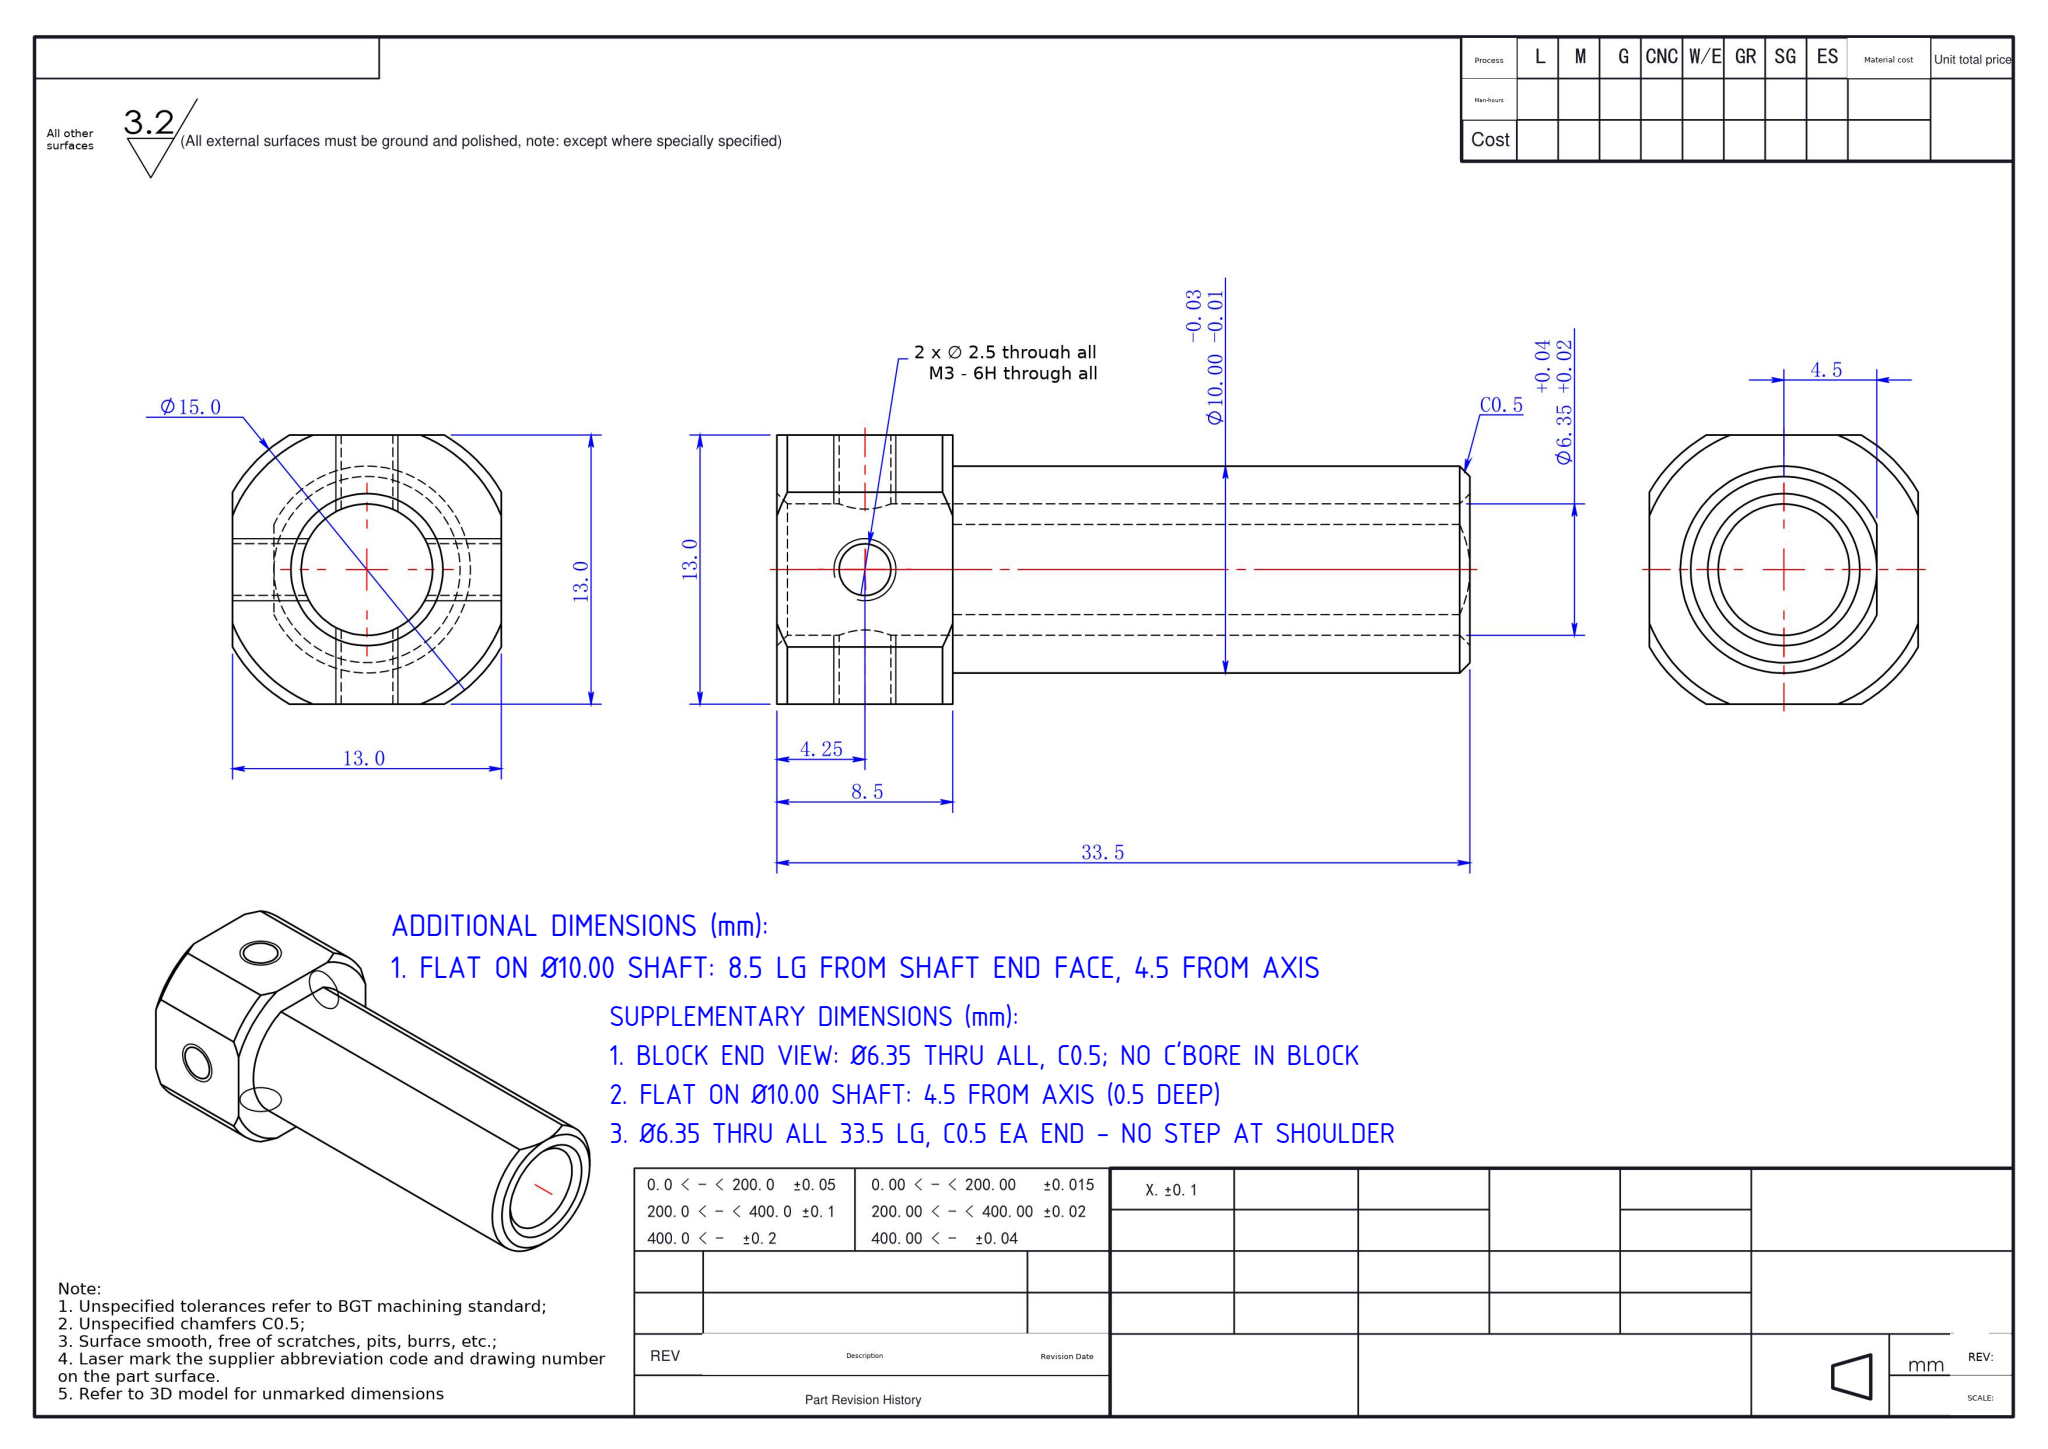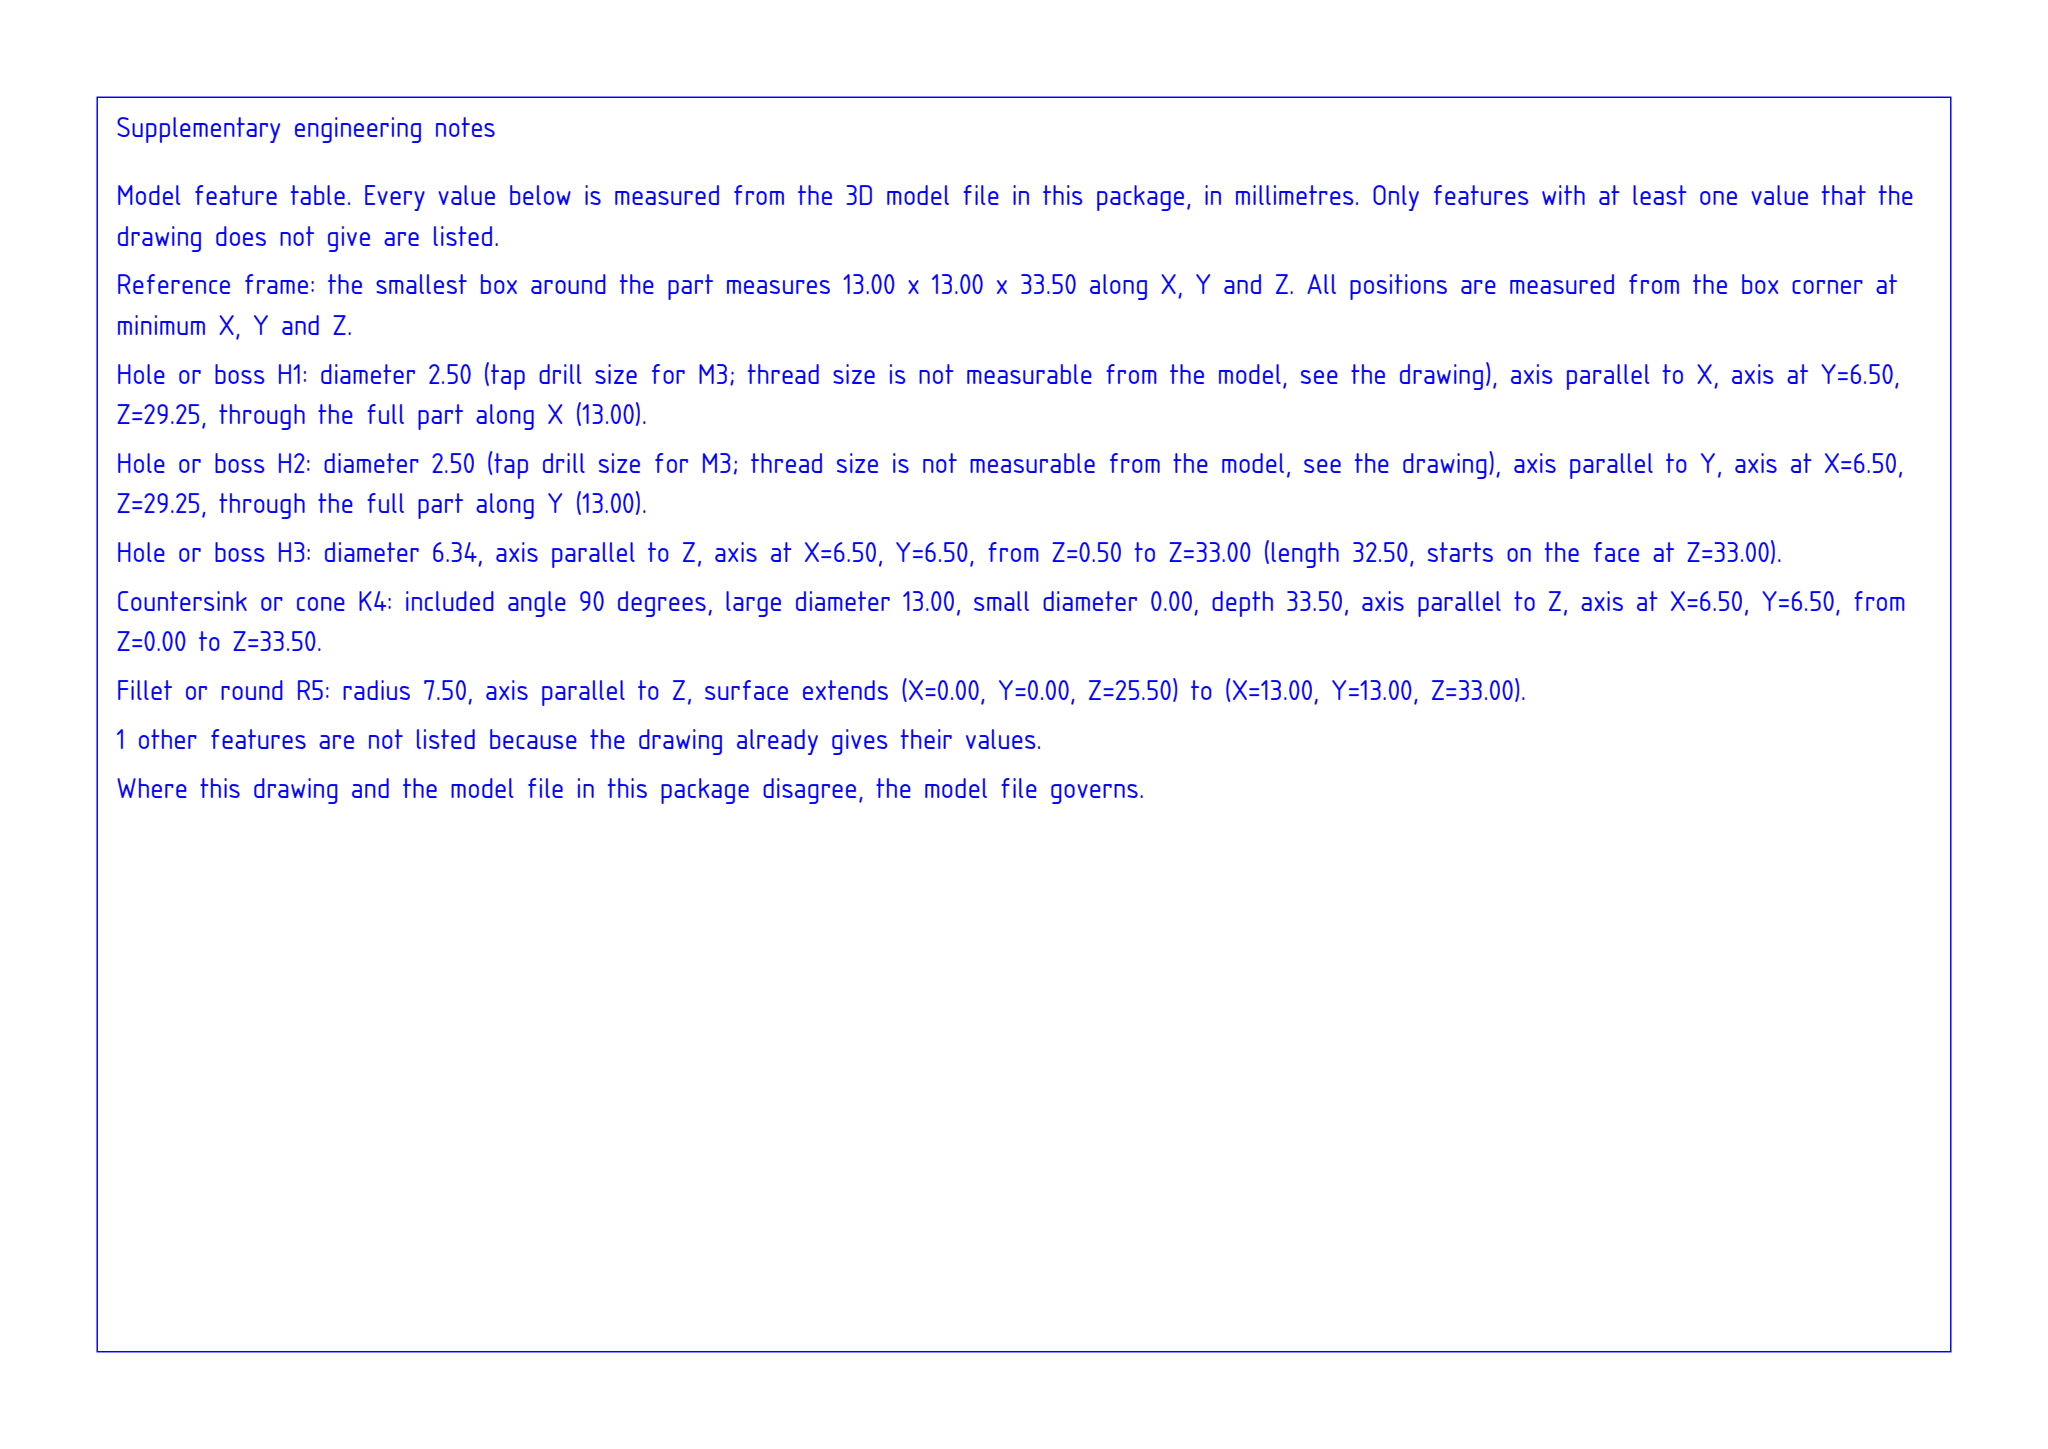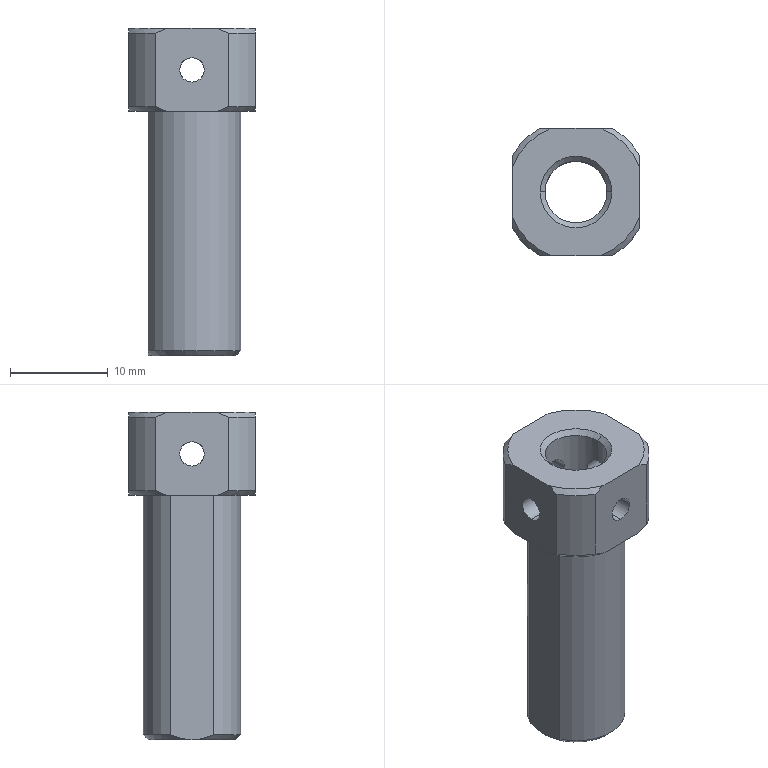Part | SolidWorks | mm | 1 solid | 38 faces | box 13 x 13 x 33.5 mm | volume 2116 mm3 | cylinder 16 | cone 14 | plane 8 | commonest cylinder face diameters 2.5 x8 15 x4 6.35 x2 10 x2